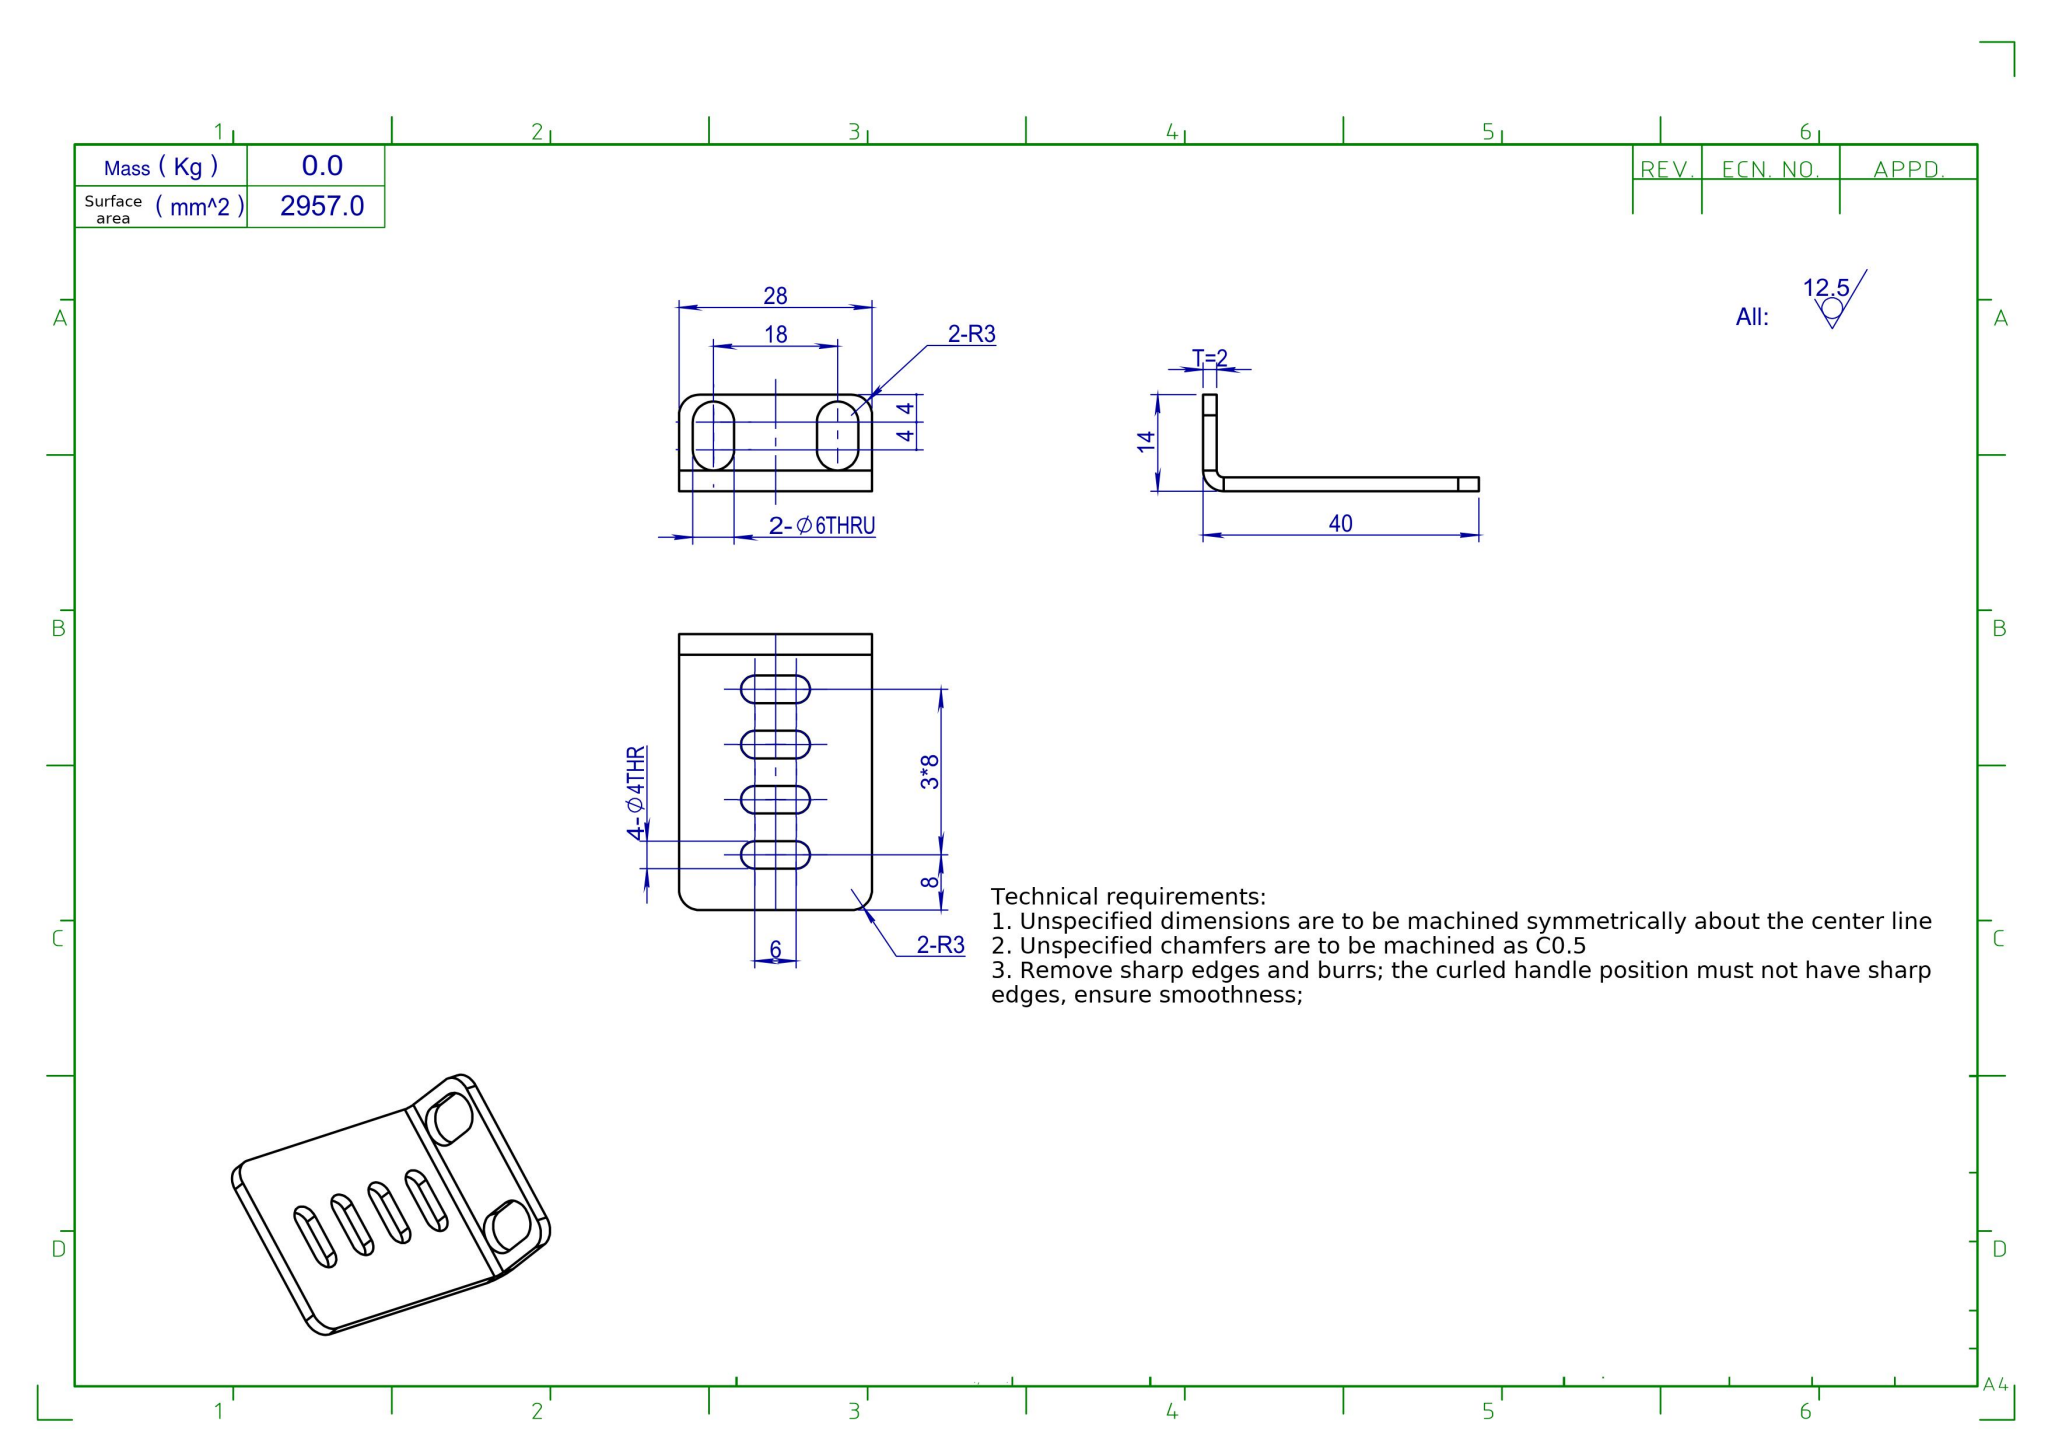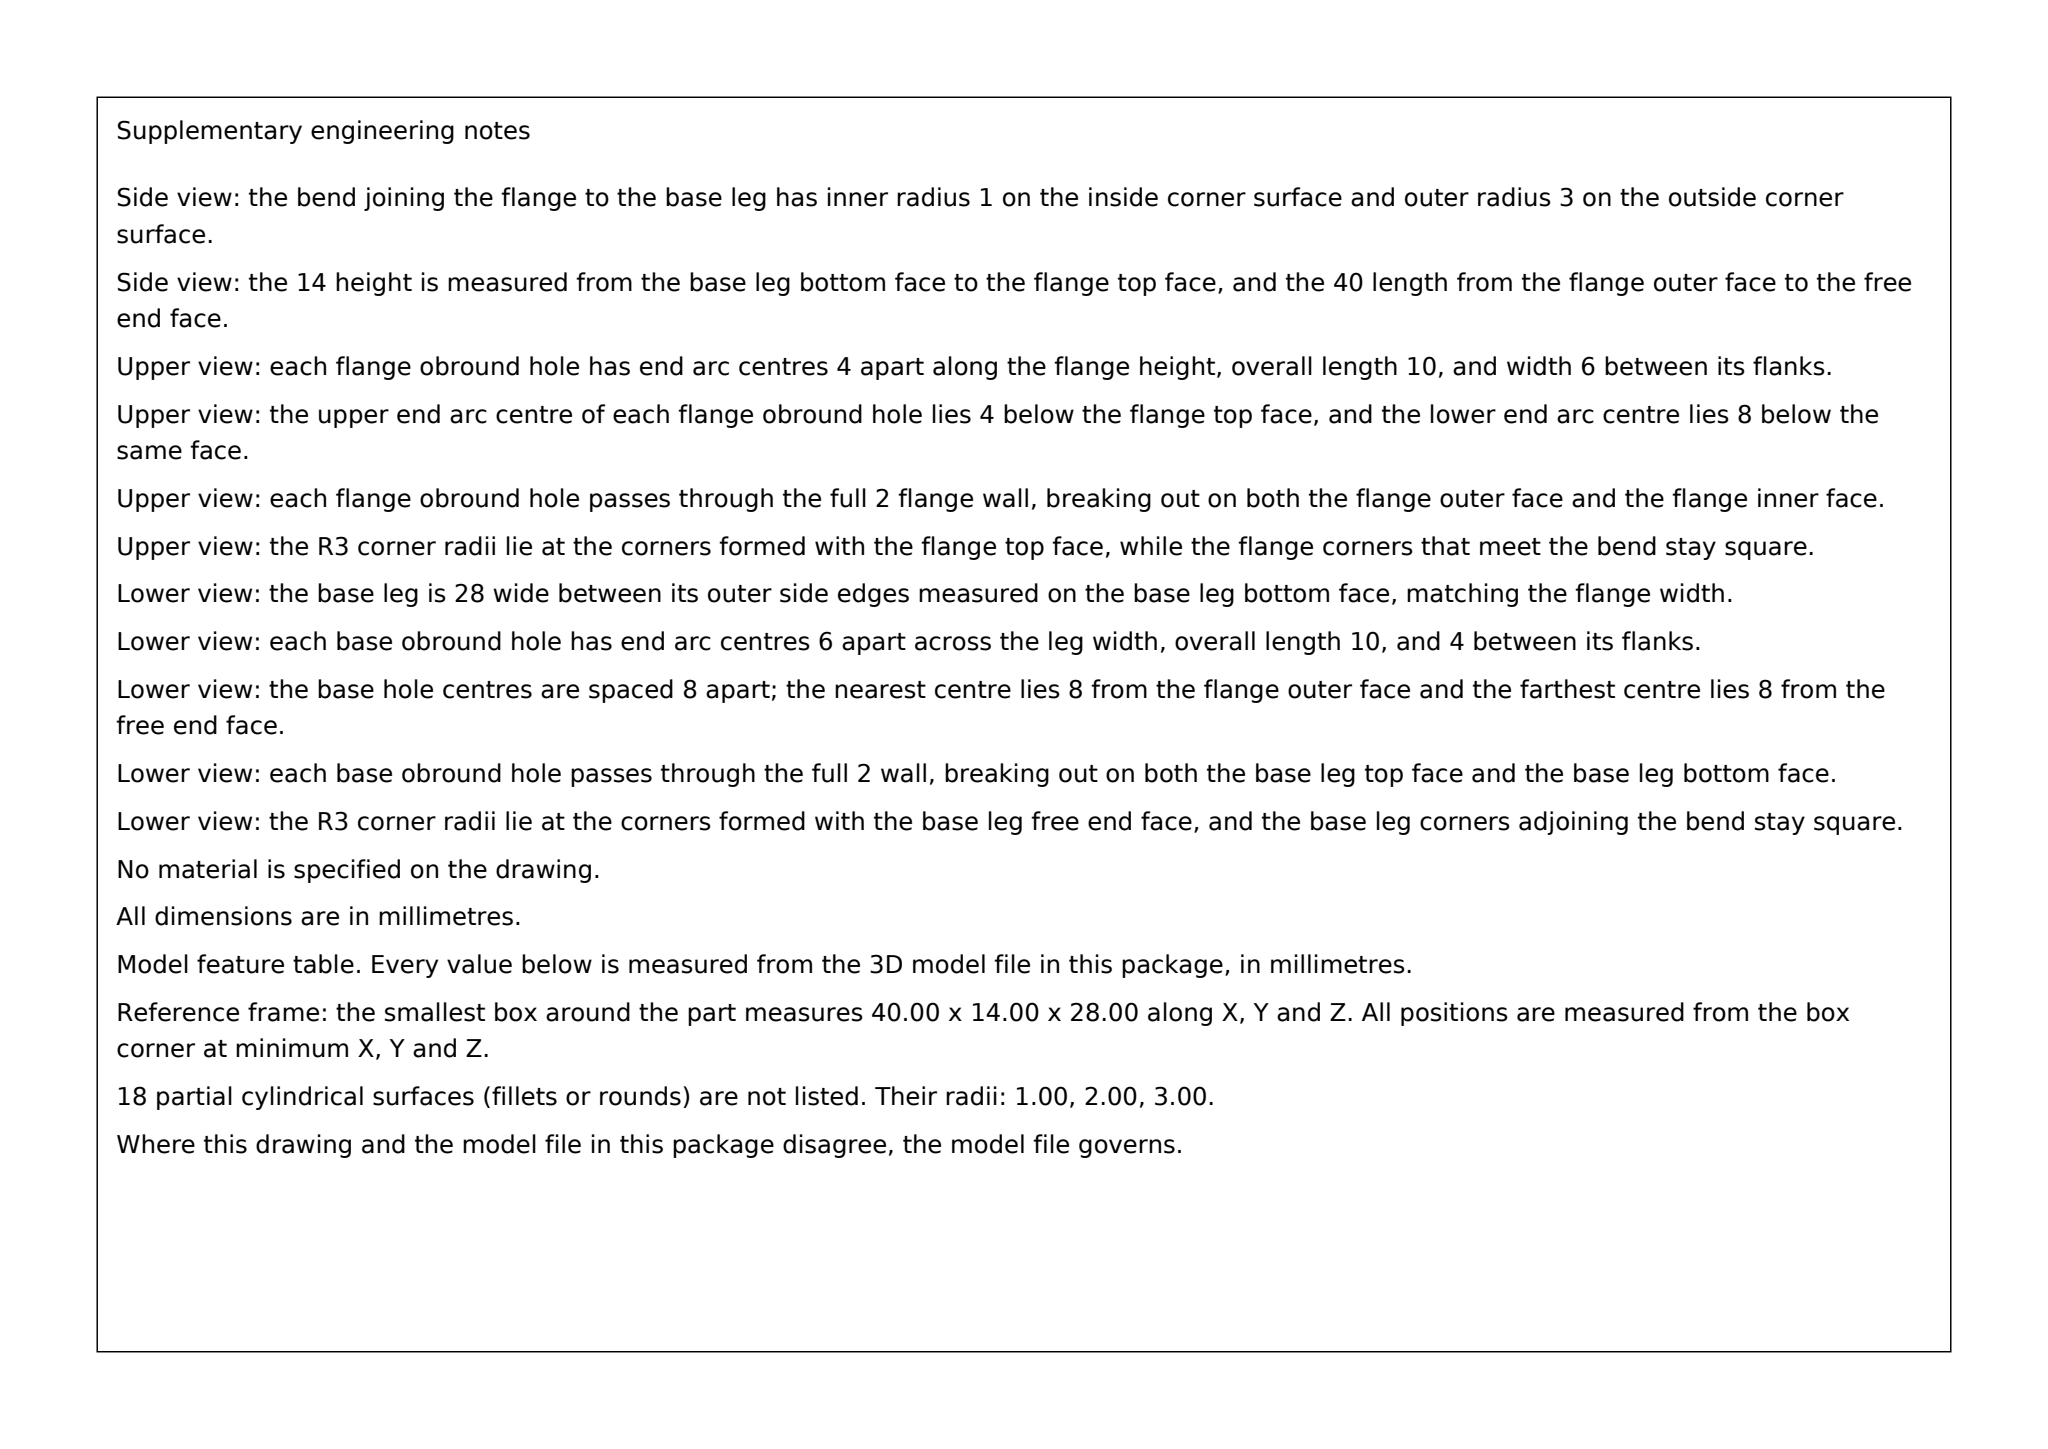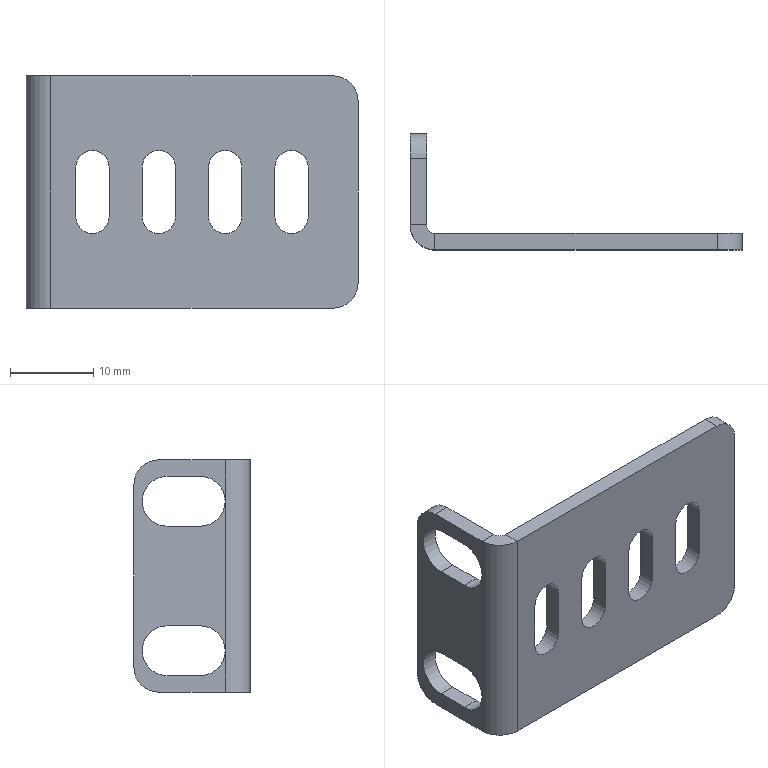Part | SolidWorks | mm | 1 solid | 46 faces | box 40 x 14 x 28 mm | volume 2347 mm3 | plane 24 | cylinder 22 | commonest cylinder face diameters 4 x12 6 x9 2 x1
Drawing notes:
2-Ø6 THRU SLOTS 10 LG (6 WD x 4 ARC C-C) IN T=2 FLANGE, ARC CL 6 & 10 FROM BASE | from the solid: Ø6 cyls axis x, len 2, planes x=0/x=2; arc centres (y6,z5)-(y10,z5) and (y6,z23)-(y10,z23)